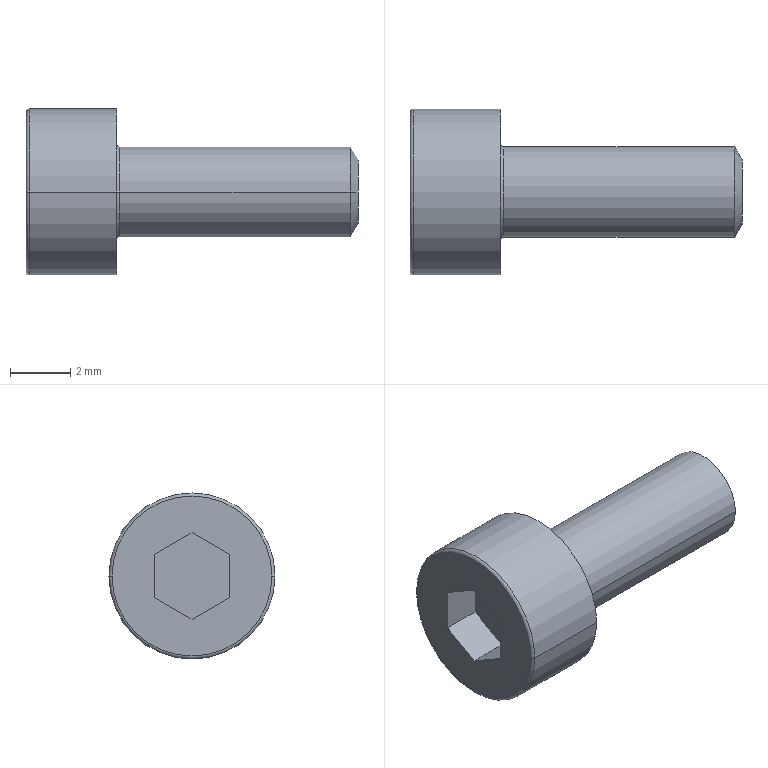Component | NX | GB_T_70_1_2008_HEX_SOCKET_CAP_SCREW_M3X8 | 1 solid | 20 faces | volume 120 mm3 | plane 10 | torus 4 | cylinder 4 | cone 2 | commonest cylinder face diameters 5.5 x2 3 x2